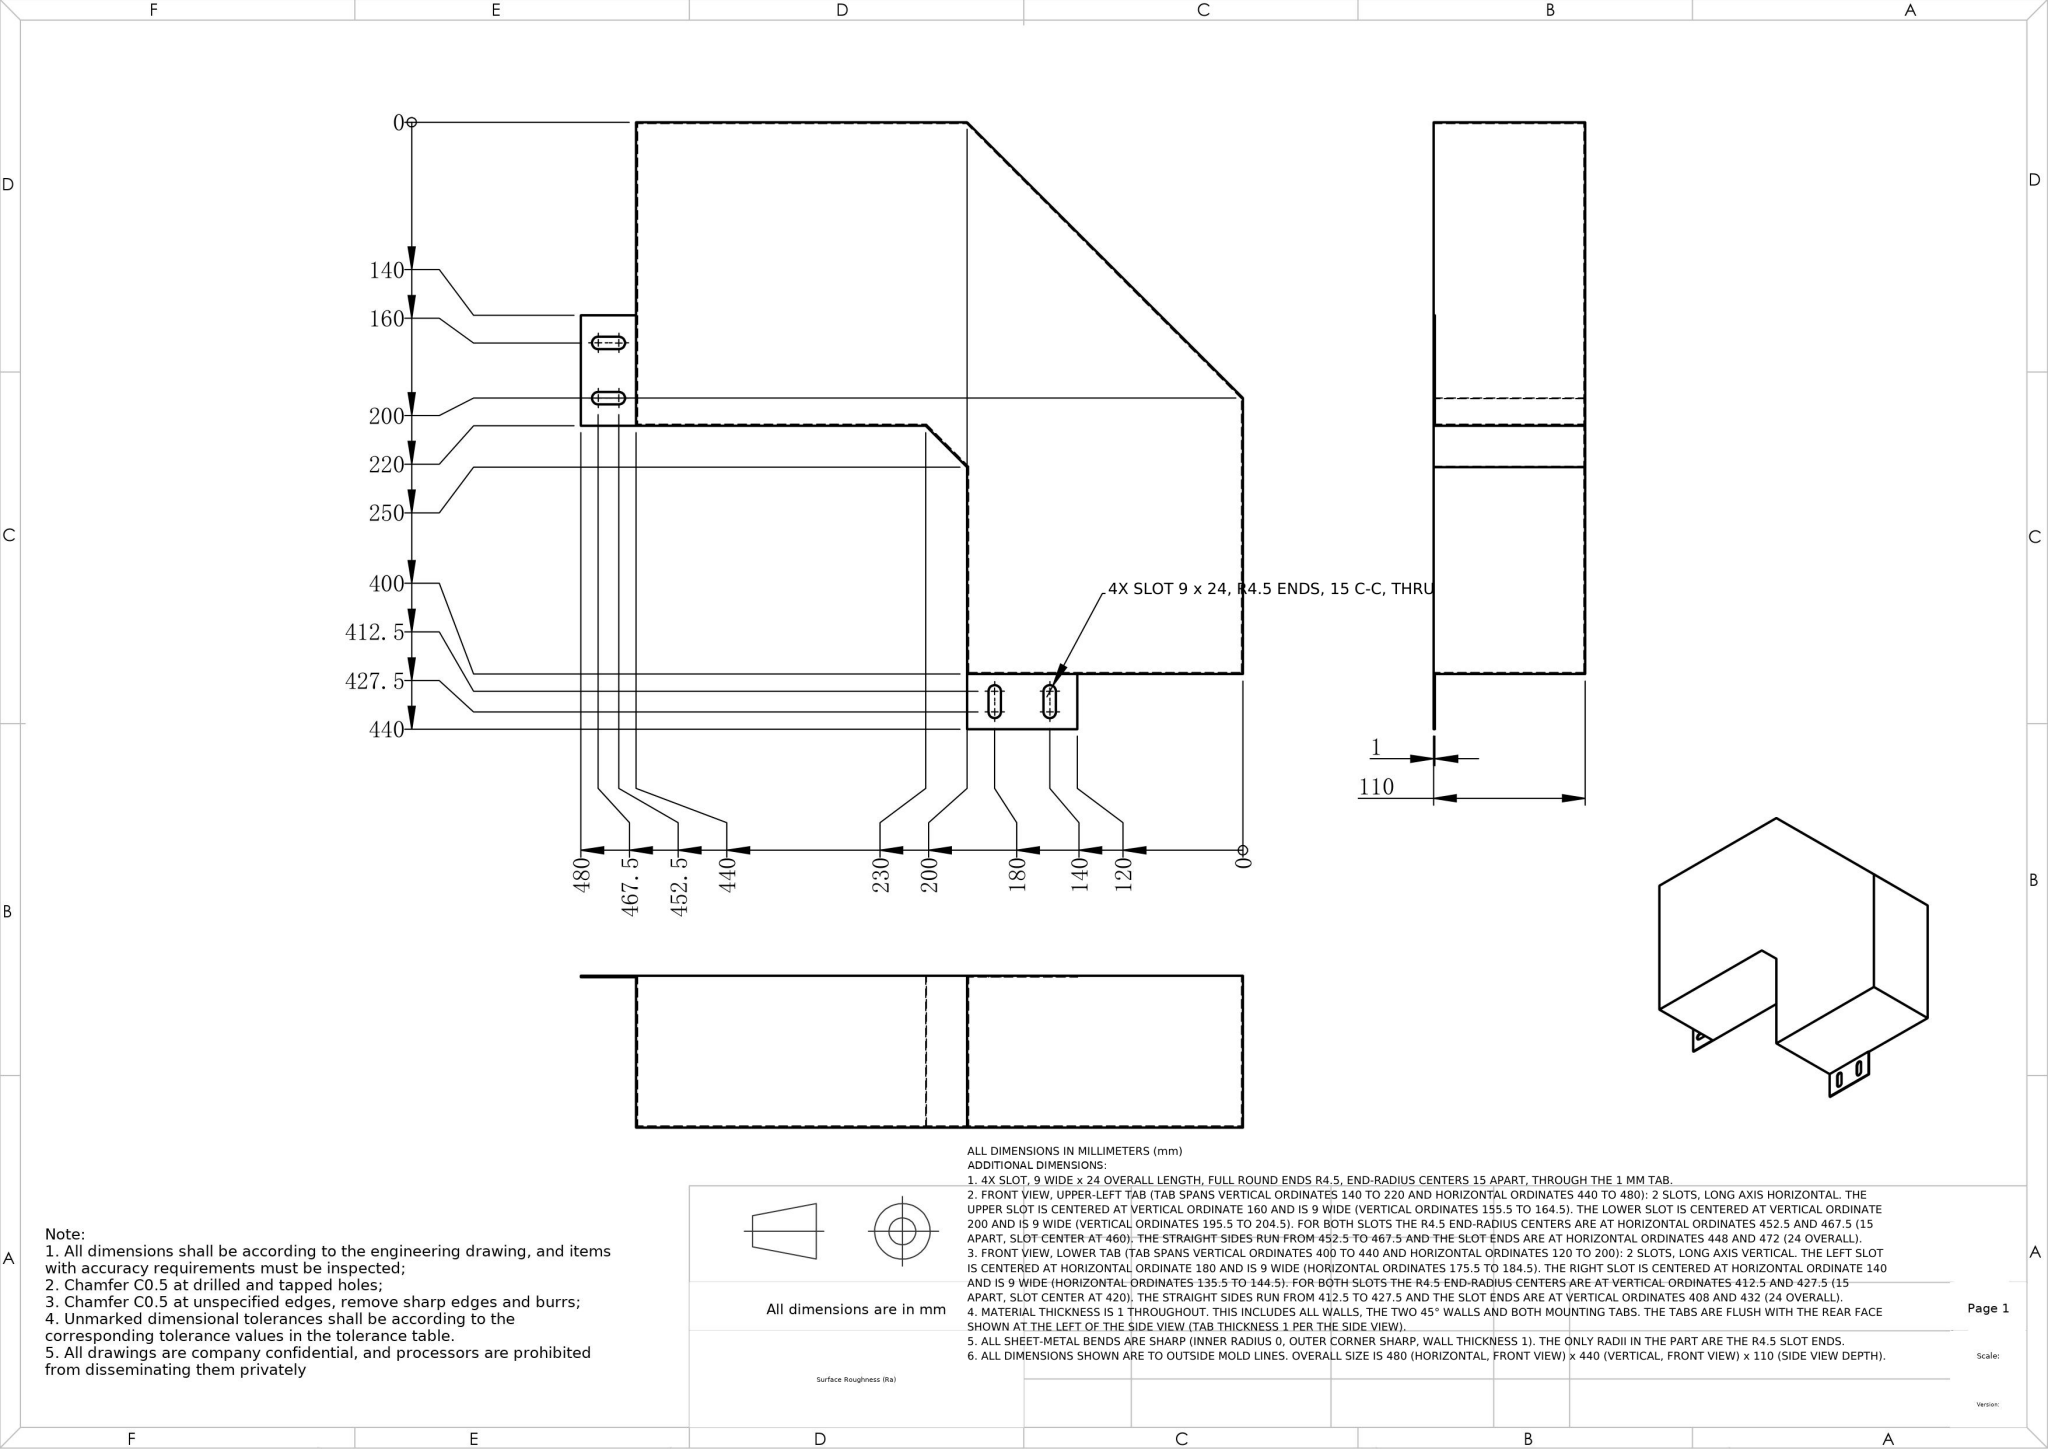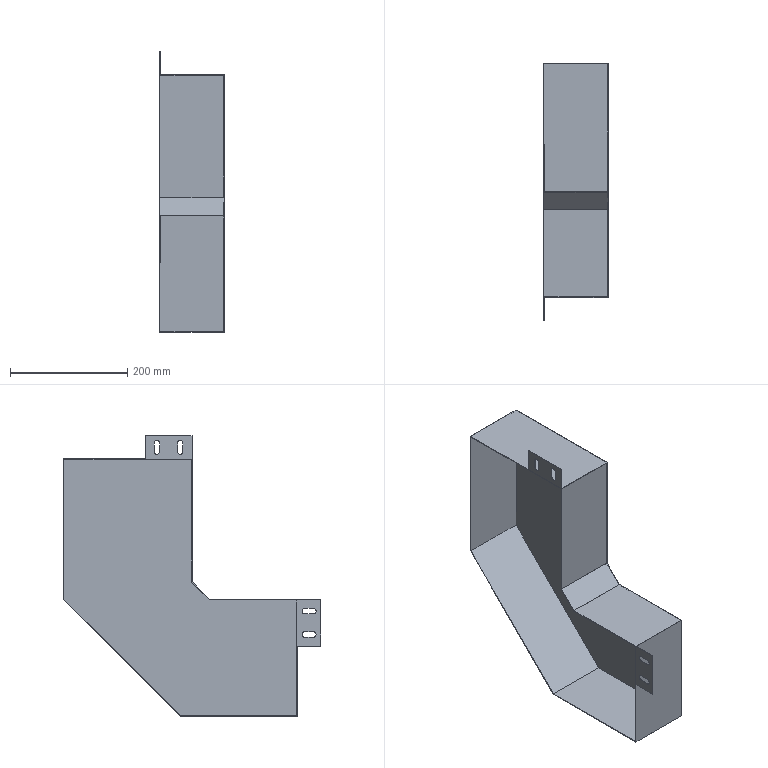Part | NX | mm | 1 solid | 43 faces | box 110 x 440 x 480 mm | volume 286854 mm3 | plane 33 | cylinder 10 | commonest cylinder face diameters 9 x10